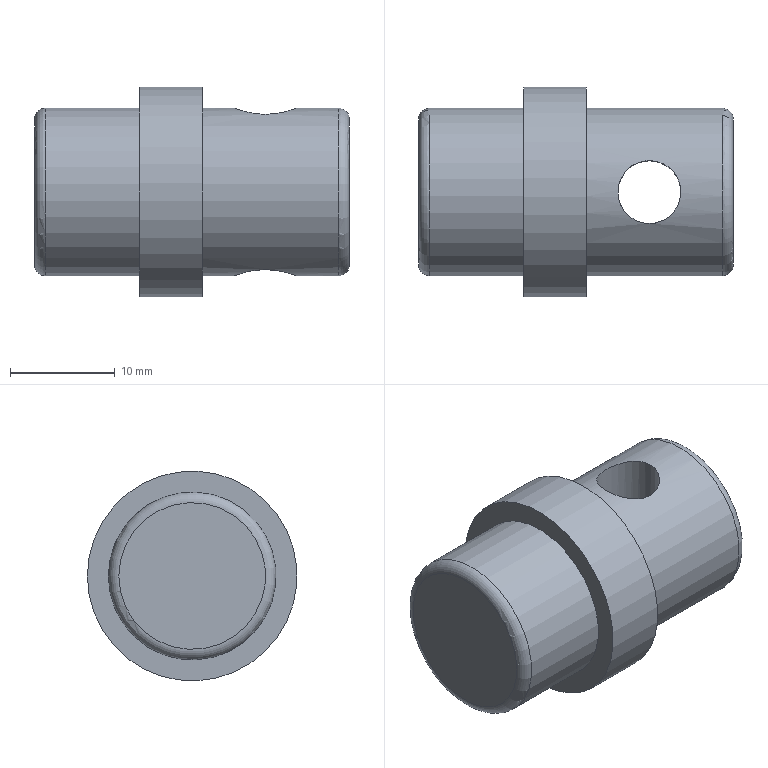Component | NX | GUIDE_BLOCK | 1 solid | 10 faces | volume 6245 mm3 | cylinder 4 | plane 4 | torus 2 | commonest cylinder face diameters 16 x2 20 x1 6 x1